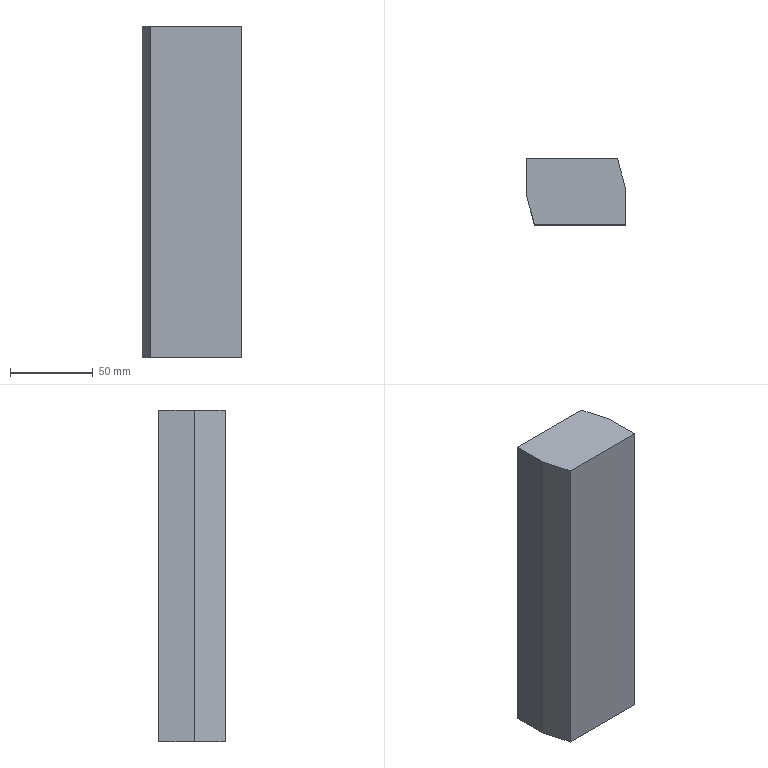Component | SolidWorks | 2023-12-12-23-1 | 1 solid | 8 faces | box 60 x 40 x 200 mm | volume 461340 mm3 | plane 8 | material AL6061
build123d program:
from build123d import *
from OCP.BRepFilletAPI import BRepFilletAPI_MakeChamfer

# Parameters (mm, degrees)
SKETCH1_R           = 14.78
BOSS_EXTRUDE1_DEPTH = 200
SKETCH2_W           = 60
SKETCH2_H           = 40
BOSS_EXTRUDE2_DEPTH = 200
CHAMFER2_SIZE       = 5
CHAMFER2_SIZE2      = 18.66


with BuildPart() as part:
    # Sketch1 → Boss-Extrude1 (new body)
    with BuildSketch(Plane.XY):
        Circle(SKETCH1_R)
    extrude(amount=BOSS_EXTRUDE1_DEPTH)

    # Sketch2 → Boss-Extrude2 (add)
    with BuildSketch(Plane(origin=(0, 0, 0), x_dir=(-1, 0, 0), z_dir=(0, 0, -1))):
        Rectangle(SKETCH2_W, SKETCH2_H)
    extrude(amount=-BOSS_EXTRUDE2_DEPTH)

    # Chamfer2: one chamfer whose edges measure the first distance from different faces: ONE call of the kernel's chamfer builder (chamfer() names one face for all edges)
    chamfer2_edges_1 = [part.edges().sort_by_distance(p)[0] for p in [
        (30, 20, 100),
    ]]
    chamfer2_side_1 = [part.faces().sort_by_distance(p)[0] for p in [
        (0, 20, 100),
    ]]
    chamfer2_edges_2 = [part.edges().sort_by_distance(p)[0] for p in [
        (-30, -20, 100),
    ]]
    chamfer2_side_2 = [part.faces().sort_by_distance(p)[0] for p in [
        (0, -20, 100),
    ]]
    chamfer2 = BRepFilletAPI_MakeChamfer(part.part.solid().wrapped)
    for e in chamfer2_edges_1:
        chamfer2.Add(CHAMFER2_SIZE, CHAMFER2_SIZE2, e.wrapped, chamfer2_side_1[0].wrapped)  # the first distance lies on this face
    for e in chamfer2_edges_2:
        chamfer2.Add(CHAMFER2_SIZE, CHAMFER2_SIZE2, e.wrapped, chamfer2_side_2[0].wrapped)  # the first distance lies on this face
    add(Compound.cast(chamfer2.Shape()), mode=Mode.REPLACE)


solid = part.part

# Placed as in the assembly
solid = solid.moved(Location((1.222, -2.867, 100), (0, 0, 0)))
STEP:
#1=COLOUR_RGB('',0.7922,0.8196,0.9333);
#2=FILL_AREA_STYLE_COLOUR('',#1);
#3=FILL_AREA_STYLE('',(#2));
#4=SURFACE_STYLE_FILL_AREA(#3);
#5=SURFACE_SIDE_STYLE('',(#4));
#6=SURFACE_STYLE_USAGE(.BOTH.,#5);
#7=PRESENTATION_STYLE_ASSIGNMENT((#6));
#8=CARTESIAN_POINT('',(1.229,-0.06012,11.811));
#9=VERTEX_POINT('',#8);
#10=CARTESIAN_POINT('',(1.229,-0.9003,11.811));
#11=VERTEX_POINT('',#10);
#12=CARTESIAN_POINT('',(1.229,0.6745,11.811));
#13=DIRECTION('',(-0.,-1.,0.));
#14=VECTOR('',#13,39.37);
#15=LINE('',#12,#14);
#16=EDGE_CURVE('',#9,#11,#15,.T.);
#17=ORIENTED_EDGE('',*,*,#16,.F.);
#18=CARTESIAN_POINT('',(1.032,0.6745,11.811));
#19=VERTEX_POINT('',#18);
#20=CARTESIAN_POINT('',(1.163,0.1859,11.811));
#21=DIRECTION('',(-0.2588,0.9659,0.));
#22=VECTOR('',#21,39.37);
#23=LINE('',#20,#22);
#24=EDGE_CURVE('',#9,#19,#23,.T.);
#25=ORIENTED_EDGE('',*,*,#24,.T.);
#26=CARTESIAN_POINT('',(-1.133,0.6745,11.811));
#27=VERTEX_POINT('',#26);
#28=CARTESIAN_POINT('',(1.229,0.6745,11.811));
#29=DIRECTION('',(1.,0.,0.));
#30=VECTOR('',#29,39.37);
#31=LINE('',#28,#30);
#32=EDGE_CURVE('',#27,#19,#31,.T.);
#33=ORIENTED_EDGE('',*,*,#32,.F.);
#34=CARTESIAN_POINT('',(-1.133,-0.1656,11.811));
#35=VERTEX_POINT('',#34);
#36=CARTESIAN_POINT('',(-1.133,0.6745,11.811));
#37=DIRECTION('',(0.,1.,0.));
#38=VECTOR('',#37,39.37);
#39=LINE('',#36,#38);
#40=EDGE_CURVE('',#35,#27,#39,.T.);
#41=ORIENTED_EDGE('',*,*,#40,.F.);
#42=CARTESIAN_POINT('',(-0.9361,-0.9003,11.811));
#43=VERTEX_POINT('',#42);
#44=CARTESIAN_POINT('',(-1.067,-0.4117,11.811));
#45=DIRECTION('',(0.2588,-0.9659,0.));
#46=VECTOR('',#45,39.37);
#47=LINE('',#44,#46);
#48=EDGE_CURVE('',#35,#43,#47,.T.);
#49=ORIENTED_EDGE('',*,*,#48,.T.);
#50=CARTESIAN_POINT('',(1.229,-0.9003,11.811));
#51=DIRECTION('',(-1.,0.,0.));
#52=VECTOR('',#51,39.37);
#53=LINE('',#50,#52);
#54=EDGE_CURVE('',#11,#43,#53,.T.);
#55=ORIENTED_EDGE('',*,*,#54,.F.);
#56=EDGE_LOOP('',(#17,#25,#33,#41,#49,#55));
#57=FACE_OUTER_BOUND('',#56,.T.);
#58=CARTESIAN_POINT('',(0.04811,-0.1129,11.811));
#59=DIRECTION('',(0.,0.,1.));
#60=DIRECTION('',(1.,0.,0.));
#61=AXIS2_PLACEMENT_3D('',#58,#59,#60);
#62=PLANE('',#61);
#63=ADVANCED_FACE('',(#57),#62,.T.);
#64=ORIENTED_EDGE('',*,*,#32,.T.);
#65=CARTESIAN_POINT('',(1.032,0.6745,3.937));
#66=VERTEX_POINT('',#65);
#67=CARTESIAN_POINT('',(1.032,0.6745,14.65));
#68=DIRECTION('',(0.,0.,-1.));
#69=VECTOR('',#68,39.37);
#70=LINE('',#67,#69);
#71=EDGE_CURVE('',#19,#66,#70,.T.);
#72=ORIENTED_EDGE('',*,*,#71,.T.);
#73=CARTESIAN_POINT('',(-1.133,0.6745,3.937));
#74=VERTEX_POINT('',#73);
#75=CARTESIAN_POINT('',(1.229,0.6745,3.937));
#76=DIRECTION('',(1.,0.,0.));
#77=VECTOR('',#76,39.37);
#78=LINE('',#75,#77);
#79=EDGE_CURVE('',#74,#66,#78,.T.);
#80=ORIENTED_EDGE('',*,*,#79,.F.);
#81=CARTESIAN_POINT('',(-1.133,0.6745,14.65));
#82=DIRECTION('',(0.,0.,-1.));
#83=VECTOR('',#82,39.37);
#84=LINE('',#81,#83);
#85=EDGE_CURVE('',#27,#74,#84,.T.);
#86=ORIENTED_EDGE('',*,*,#85,.F.);
#87=EDGE_LOOP('',(#64,#72,#80,#86));
#88=FACE_OUTER_BOUND('',#87,.T.);
#89=CARTESIAN_POINT('',(1.229,0.6745,14.65));
#90=DIRECTION('',(0.,1.,0.));
#91=DIRECTION('',(0.,0.,1.));
#92=AXIS2_PLACEMENT_3D('',#89,#90,#91);
#93=PLANE('',#92);
#94=ADVANCED_FACE('',(#88),#93,.T.);
#95=CARTESIAN_POINT('',(1.229,-0.06012,3.937));
#96=VERTEX_POINT('',#95);
#97=CARTESIAN_POINT('',(1.229,-0.9003,3.937));
#98=VERTEX_POINT('',#97);
#99=CARTESIAN_POINT('',(1.229,0.6745,3.937));
#100=DIRECTION('',(-0.,-1.,0.));
#101=VECTOR('',#100,39.37);
#102=LINE('',#99,#101);
#103=EDGE_CURVE('',#96,#98,#102,.T.);
#104=ORIENTED_EDGE('',*,*,#103,.F.);
#105=CARTESIAN_POINT('',(1.229,-0.06012,14.65));
#106=DIRECTION('',(0.,0.,1.));
#107=VECTOR('',#106,39.37);
#108=LINE('',#105,#107);
#109=EDGE_CURVE('',#96,#9,#108,.T.);
#110=ORIENTED_EDGE('',*,*,#109,.T.);
#111=ORIENTED_EDGE('',*,*,#16,.T.);
#112=CARTESIAN_POINT('',(1.229,-0.9003,14.65));
#113=DIRECTION('',(0.,0.,-1.));
#114=VECTOR('',#113,39.37);
#115=LINE('',#112,#114);
#116=EDGE_CURVE('',#11,#98,#115,.T.);
#117=ORIENTED_EDGE('',*,*,#116,.T.);
#118=EDGE_LOOP('',(#104,#110,#111,#117));
#119=FACE_OUTER_BOUND('',#118,.T.);
#120=CARTESIAN_POINT('',(1.229,0.6745,14.65));
#121=DIRECTION('',(1.,-0.,0.));
#122=DIRECTION('',(0.,1.,0.));
#123=AXIS2_PLACEMENT_3D('',#120,#121,#122);
#124=PLANE('',#123);
#125=ADVANCED_FACE('',(#119),#124,.T.);
#126=ORIENTED_EDGE('',*,*,#54,.T.);
#127=CARTESIAN_POINT('',(-0.9361,-0.9003,3.937));
#128=VERTEX_POINT('',#127);
#129=CARTESIAN_POINT('',(-0.9361,-0.9003,14.65));
#130=DIRECTION('',(0.,0.,-1.));
#131=VECTOR('',#130,39.37);
#132=LINE('',#129,#131);
#133=EDGE_CURVE('',#43,#128,#132,.T.);
#134=ORIENTED_EDGE('',*,*,#133,.T.);
#135=CARTESIAN_POINT('',(1.229,-0.9003,3.937));
#136=DIRECTION('',(-1.,0.,0.));
#137=VECTOR('',#136,39.37);
#138=LINE('',#135,#137);
#139=EDGE_CURVE('',#98,#128,#138,.T.);
#140=ORIENTED_EDGE('',*,*,#139,.F.);
#141=ORIENTED_EDGE('',*,*,#116,.F.);
#142=EDGE_LOOP('',(#126,#134,#140,#141));
#143=FACE_OUTER_BOUND('',#142,.T.);
#144=CARTESIAN_POINT('',(1.229,-0.9003,14.65));
#145=DIRECTION('',(0.,-1.,0.));
#146=DIRECTION('',(0.,0.,-1.));
#147=AXIS2_PLACEMENT_3D('',#144,#145,#146);
#148=PLANE('',#147);
#149=ADVANCED_FACE('',(#143),#148,.T.);
#150=CARTESIAN_POINT('',(-1.133,-0.1656,3.937));
#151=VERTEX_POINT('',#150);
#152=CARTESIAN_POINT('',(-1.133,0.6745,3.937));
#153=DIRECTION('',(0.,1.,0.));
#154=VECTOR('',#153,39.37);
#155=LINE('',#152,#154);
#156=EDGE_CURVE('',#151,#74,#155,.T.);
#157=ORIENTED_EDGE('',*,*,#156,.F.);
#158=CARTESIAN_POINT('',(-1.133,-0.1656,14.65));
#159=DIRECTION('',(0.,0.,1.));
#160=VECTOR('',#159,39.37);
#161=LINE('',#158,#160);
#162=EDGE_CURVE('',#151,#35,#161,.T.);
#163=ORIENTED_EDGE('',*,*,#162,.T.);
#164=ORIENTED_EDGE('',*,*,#40,.T.);
#165=ORIENTED_EDGE('',*,*,#85,.T.);
#166=EDGE_LOOP('',(#157,#163,#164,#165));
#167=FACE_OUTER_BOUND('',#166,.T.);
#168=CARTESIAN_POINT('',(-1.133,0.6745,14.65));
#169=DIRECTION('',(-1.,0.,0.));
#170=DIRECTION('',(-0.,-1.,0.));
#171=AXIS2_PLACEMENT_3D('',#168,#169,#170);
#172=PLANE('',#171);
#173=ADVANCED_FACE('',(#167),#172,.T.);
#174=ORIENTED_EDGE('',*,*,#79,.T.);
#175=CARTESIAN_POINT('',(1.032,0.6745,3.937));
#176=DIRECTION('',(0.2588,-0.9659,0.));
#177=VECTOR('',#176,39.37);
#178=LINE('',#175,#177);
#179=EDGE_CURVE('',#66,#96,#178,.T.);
#180=ORIENTED_EDGE('',*,*,#179,.T.);
#181=ORIENTED_EDGE('',*,*,#103,.T.);
#182=ORIENTED_EDGE('',*,*,#139,.T.);
#183=CARTESIAN_POINT('',(-0.9361,-0.9003,3.937));
#184=DIRECTION('',(-0.2588,0.9659,0.));
#185=VECTOR('',#184,39.37);
#186=LINE('',#183,#185);
#187=EDGE_CURVE('',#128,#151,#186,.T.);
#188=ORIENTED_EDGE('',*,*,#187,.T.);
#189=ORIENTED_EDGE('',*,*,#156,.T.);
#190=EDGE_LOOP('',(#174,#180,#181,#182,#188,#189));
#191=FACE_OUTER_BOUND('',#190,.T.);
#192=CARTESIAN_POINT('',(0.04811,-0.1129,3.937));
#193=DIRECTION('',(0.,0.,1.));
#194=DIRECTION('',(1.,0.,0.));
#195=AXIS2_PLACEMENT_3D('',#192,#193,#194);
#196=PLANE('',#195);
#197=ADVANCED_FACE('',(#191),#196,.F.);
#198=ORIENTED_EDGE('',*,*,#24,.F.);
#199=ORIENTED_EDGE('',*,*,#109,.F.);
#200=ORIENTED_EDGE('',*,*,#179,.F.);
#201=ORIENTED_EDGE('',*,*,#71,.F.);
#202=EDGE_LOOP('',(#198,#199,#200,#201));
#203=FACE_OUTER_BOUND('',#202,.T.);
#204=CARTESIAN_POINT('',(1.032,0.6745,14.65));
#205=DIRECTION('',(-0.9659,-0.2588,0.));
#206=DIRECTION('',(0.,0.,-1.));
#207=AXIS2_PLACEMENT_3D('',#204,#205,#206);
#208=PLANE('',#207);
#209=ADVANCED_FACE('',(#203),#208,.F.);
#210=ORIENTED_EDGE('',*,*,#48,.F.);
#211=ORIENTED_EDGE('',*,*,#162,.F.);
#212=ORIENTED_EDGE('',*,*,#187,.F.);
#213=ORIENTED_EDGE('',*,*,#133,.F.);
#214=EDGE_LOOP('',(#210,#211,#212,#213));
#215=FACE_OUTER_BOUND('',#214,.T.);
#216=CARTESIAN_POINT('',(-0.9361,-0.9003,14.65));
#217=DIRECTION('',(0.9659,0.2588,0.));
#218=DIRECTION('',(0.,0.,-1.));
#219=AXIS2_PLACEMENT_3D('',#216,#217,#218);
#220=PLANE('',#219);
#221=ADVANCED_FACE('',(#215),#220,.F.);
#222=CLOSED_SHELL('',(#63,#94,#125,#149,#173,#197,#209,#221));
#223=MANIFOLD_SOLID_BREP('',#222);
#224=STYLED_ITEM('',(#7),#223);
#225=(LENGTH_UNIT()NAMED_UNIT(*)SI_UNIT($,.METRE.));
#226=LENGTH_MEASURE_WITH_UNIT(LENGTH_MEASURE(0.0254),#225);
#227=DIMENSIONAL_EXPONENTS(1.,0.,0.,0.,0.,0.,0.);
#228=(CONVERSION_BASED_UNIT('',#226)LENGTH_UNIT()NAMED_UNIT(#227));
#229=UNCERTAINTY_MEASURE_WITH_UNIT(LENGTH_MEASURE(0.00001),#228,'','');
#230=(NAMED_UNIT(*)PLANE_ANGLE_UNIT()SI_UNIT($,.RADIAN.));
#231=(NAMED_UNIT(*)SI_UNIT($,.STERADIAN.)SOLID_ANGLE_UNIT());
#232=(GEOMETRIC_REPRESENTATION_CONTEXT(3)GLOBAL_UNCERTAINTY_ASSIGNED_CONTEXT((#229))GLOBAL_UNIT_ASSIGNED_CONTEXT((#228,#230,#231))REPRESENTATION_CONTEXT('',''));
#233=MECHANICAL_DESIGN_GEOMETRIC_PRESENTATION_REPRESENTATION('',(#224),#232);
#234=CARTESIAN_POINT('',(0.,0.,0.));
#235=DIRECTION('',(0.,0.,1.));
#236=DIRECTION('',(1.,0.,0.));
#237=AXIS2_PLACEMENT_3D('',#234,#235,#236);
#238=(LENGTH_UNIT()NAMED_UNIT(*)SI_UNIT($,.METRE.));
#239=LENGTH_MEASURE_WITH_UNIT(LENGTH_MEASURE(0.0254),#238);
#240=DIMENSIONAL_EXPONENTS(1.,0.,0.,0.,0.,0.,0.);
#241=(CONVERSION_BASED_UNIT('',#239)LENGTH_UNIT()NAMED_UNIT(#240));
#242=UNCERTAINTY_MEASURE_WITH_UNIT(LENGTH_MEASURE(0.00001),#241,'','');
#243=(NAMED_UNIT(*)PLANE_ANGLE_UNIT()SI_UNIT($,.RADIAN.));
#244=(NAMED_UNIT(*)SI_UNIT($,.STERADIAN.)SOLID_ANGLE_UNIT());
#245=(GEOMETRIC_REPRESENTATION_CONTEXT(3)GLOBAL_UNCERTAINTY_ASSIGNED_CONTEXT((#242))GLOBAL_UNIT_ASSIGNED_CONTEXT((#241,#243,#244))REPRESENTATION_CONTEXT('',''));
#246=ADVANCED_BREP_SHAPE_REPRESENTATION('',(#223,#237),#245);
#247=PRESENTATION_LAYER_ASSIGNMENT('','',(#224));